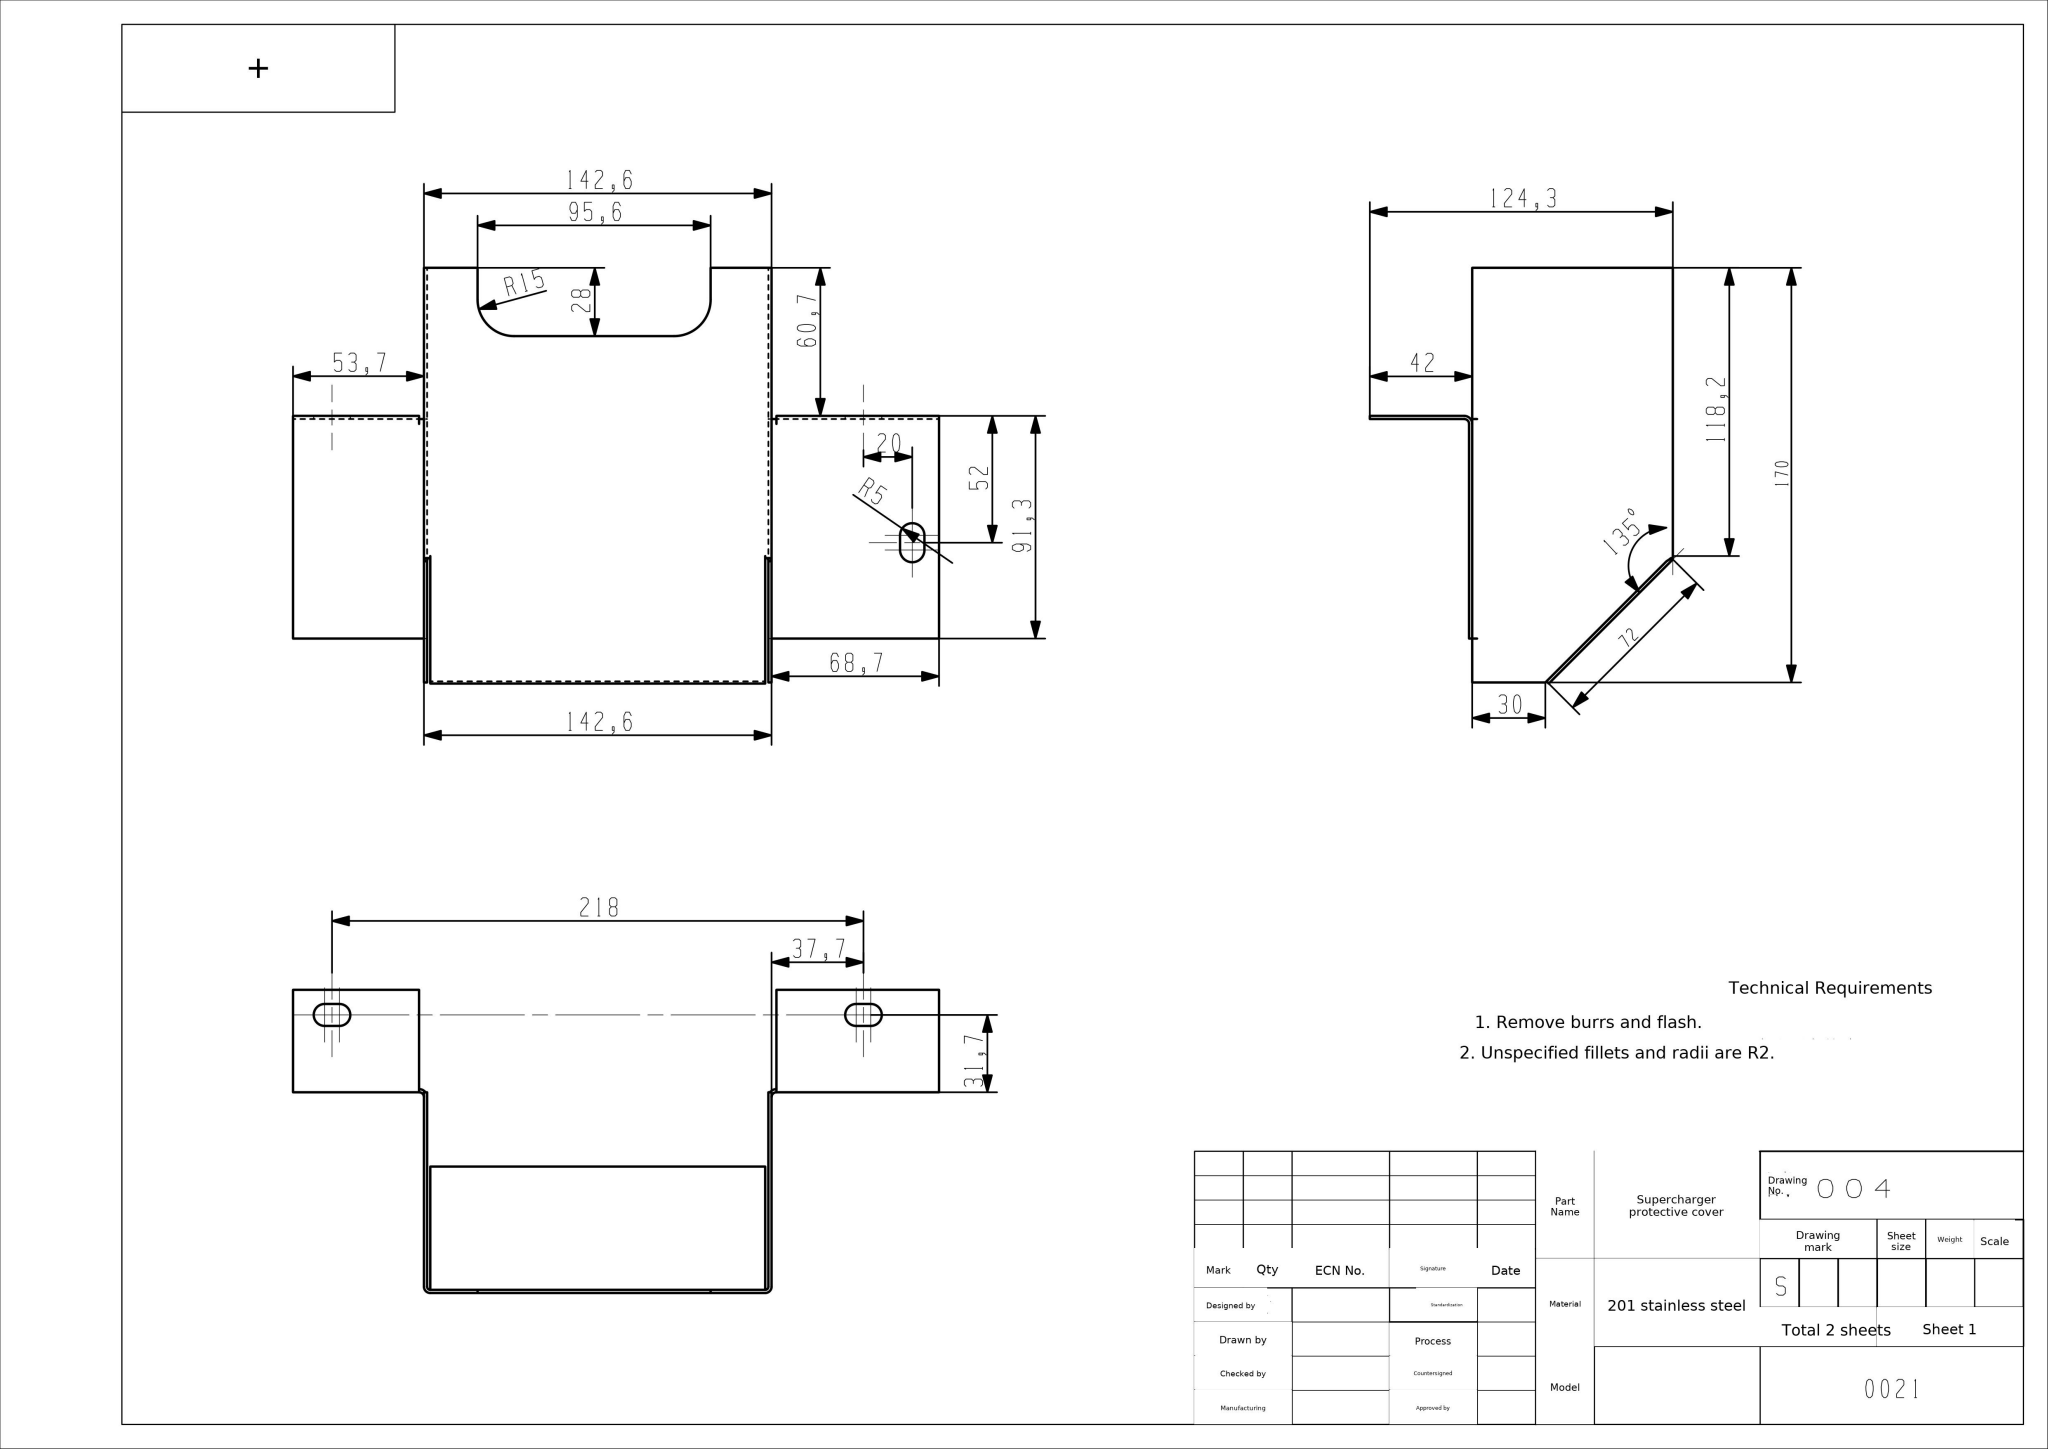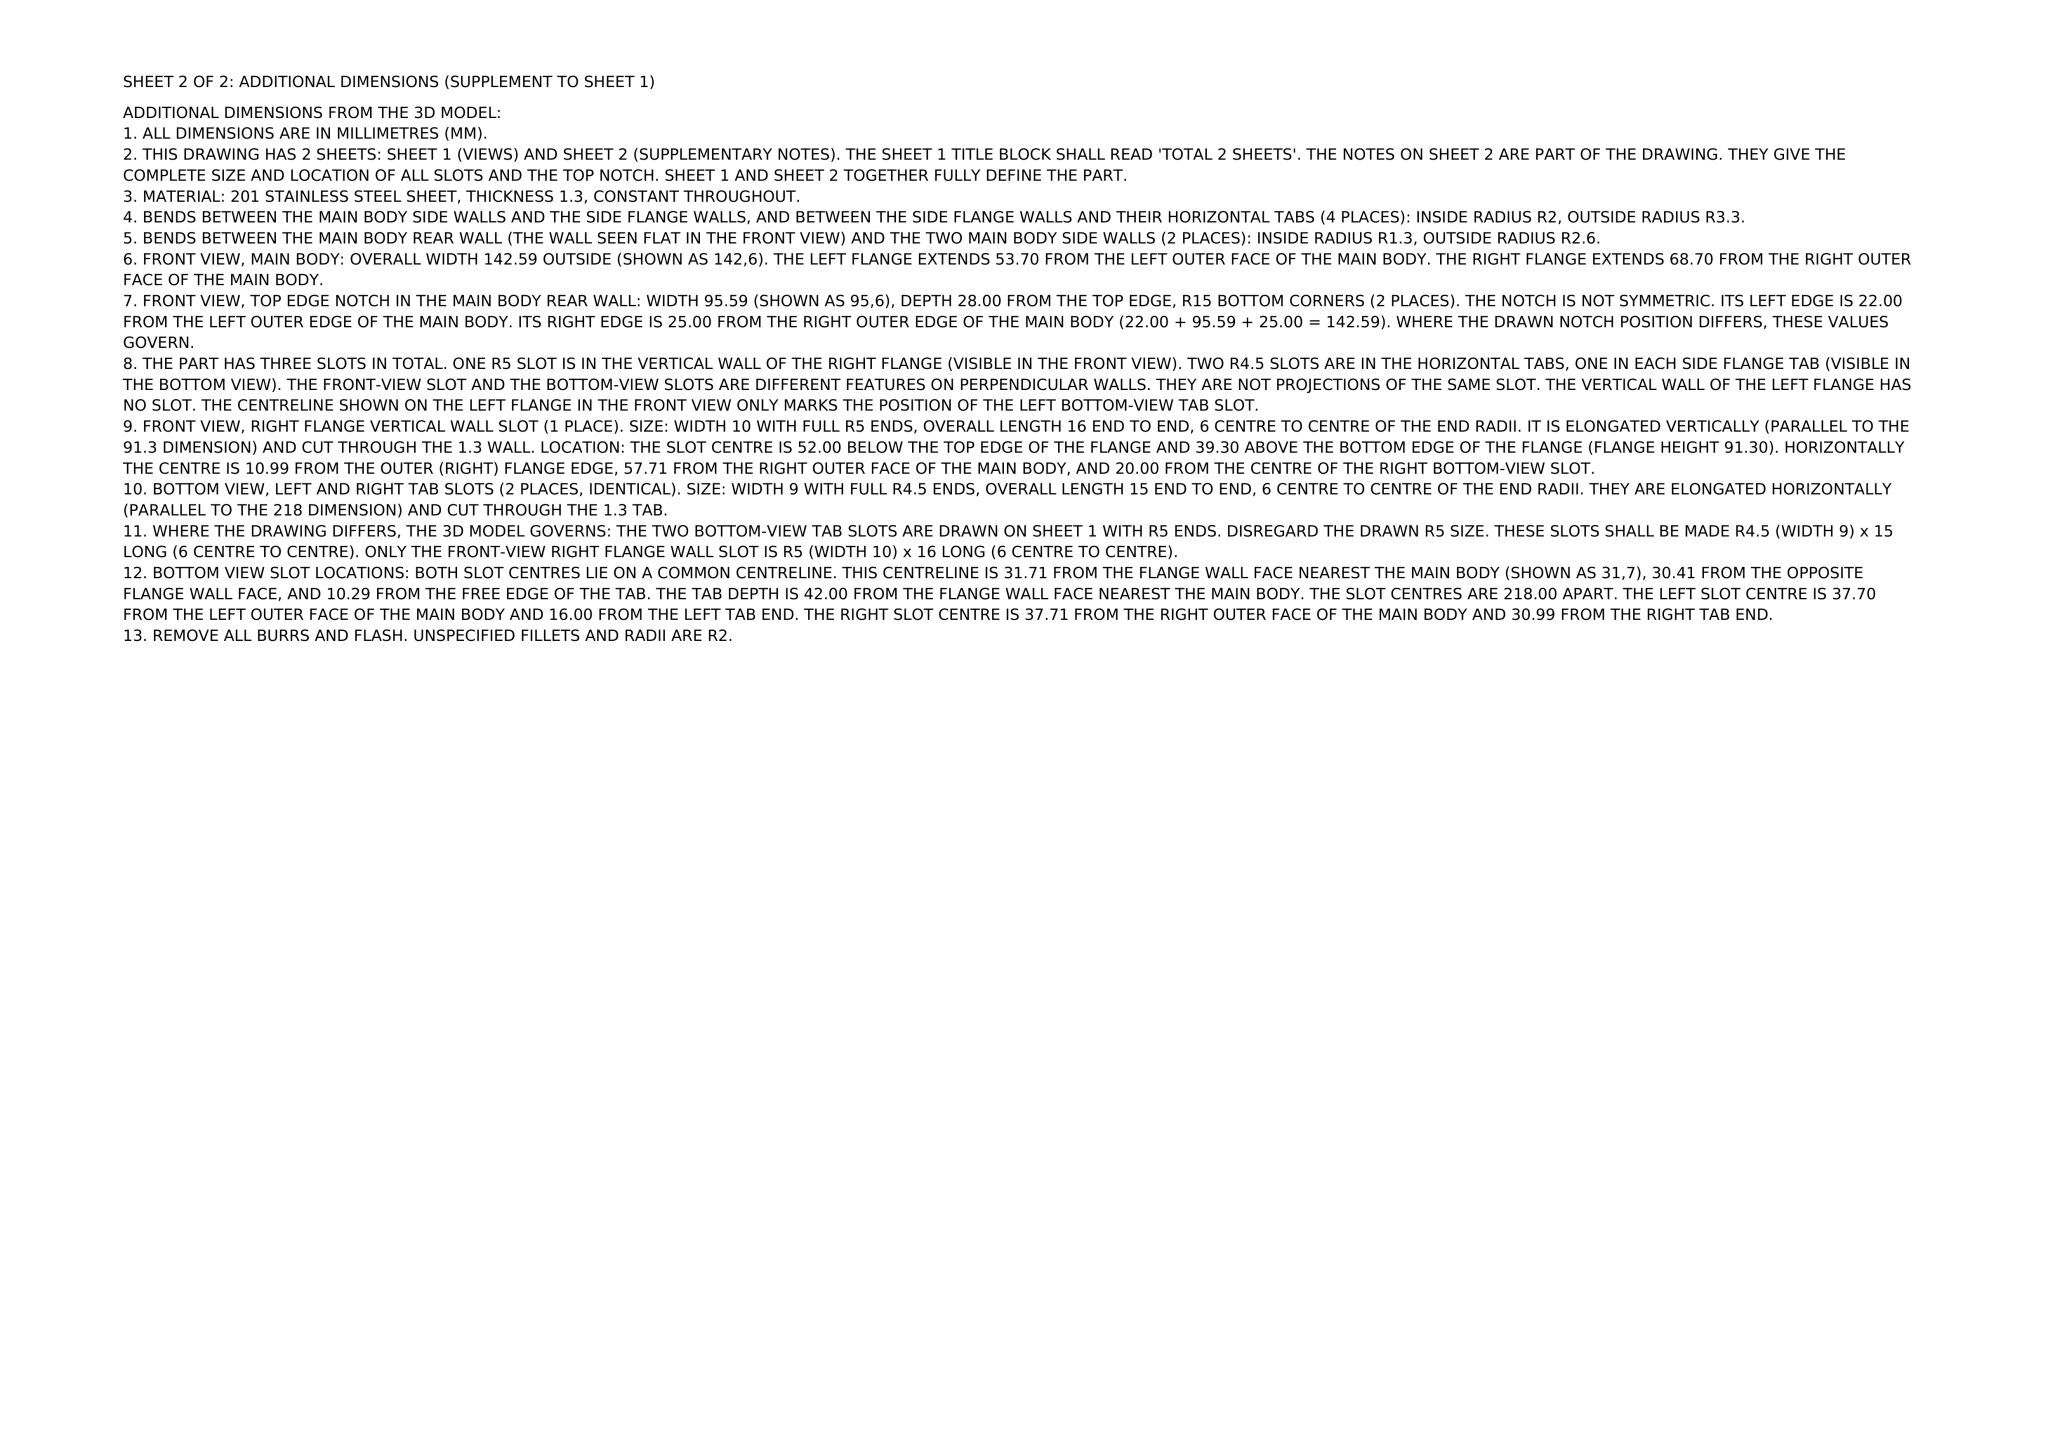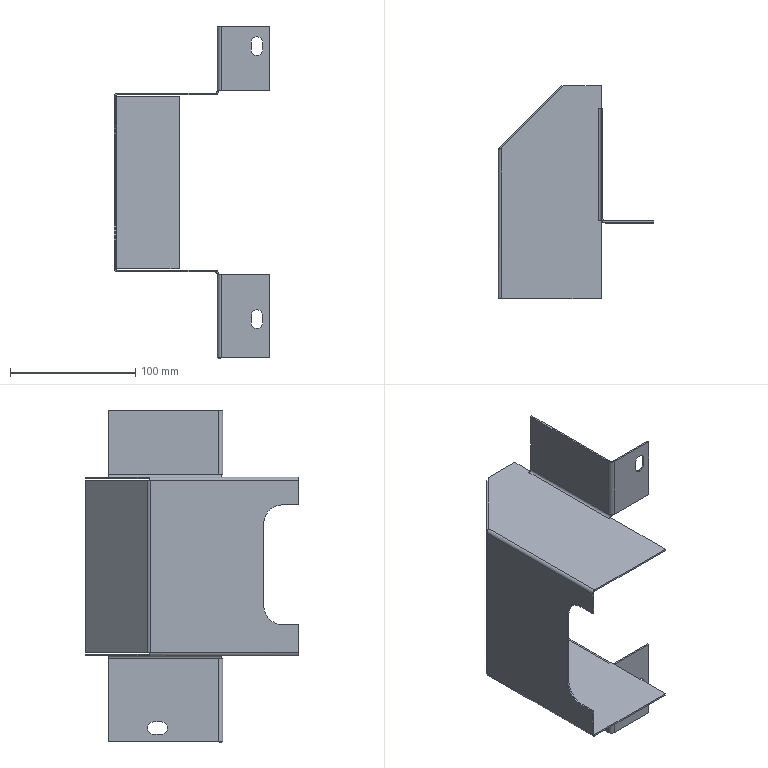Part | NX | mm | 1 solid | 90 faces | box 124.29 x 170.45 x 264.99 mm | volume 83865 mm3 | plane 66 | cylinder 22 | spline 2 | commonest cylinder face diameters 6.6 x5 4 x5 9 x4 5.2 x2 2.6 x2 30 x2 10 x2